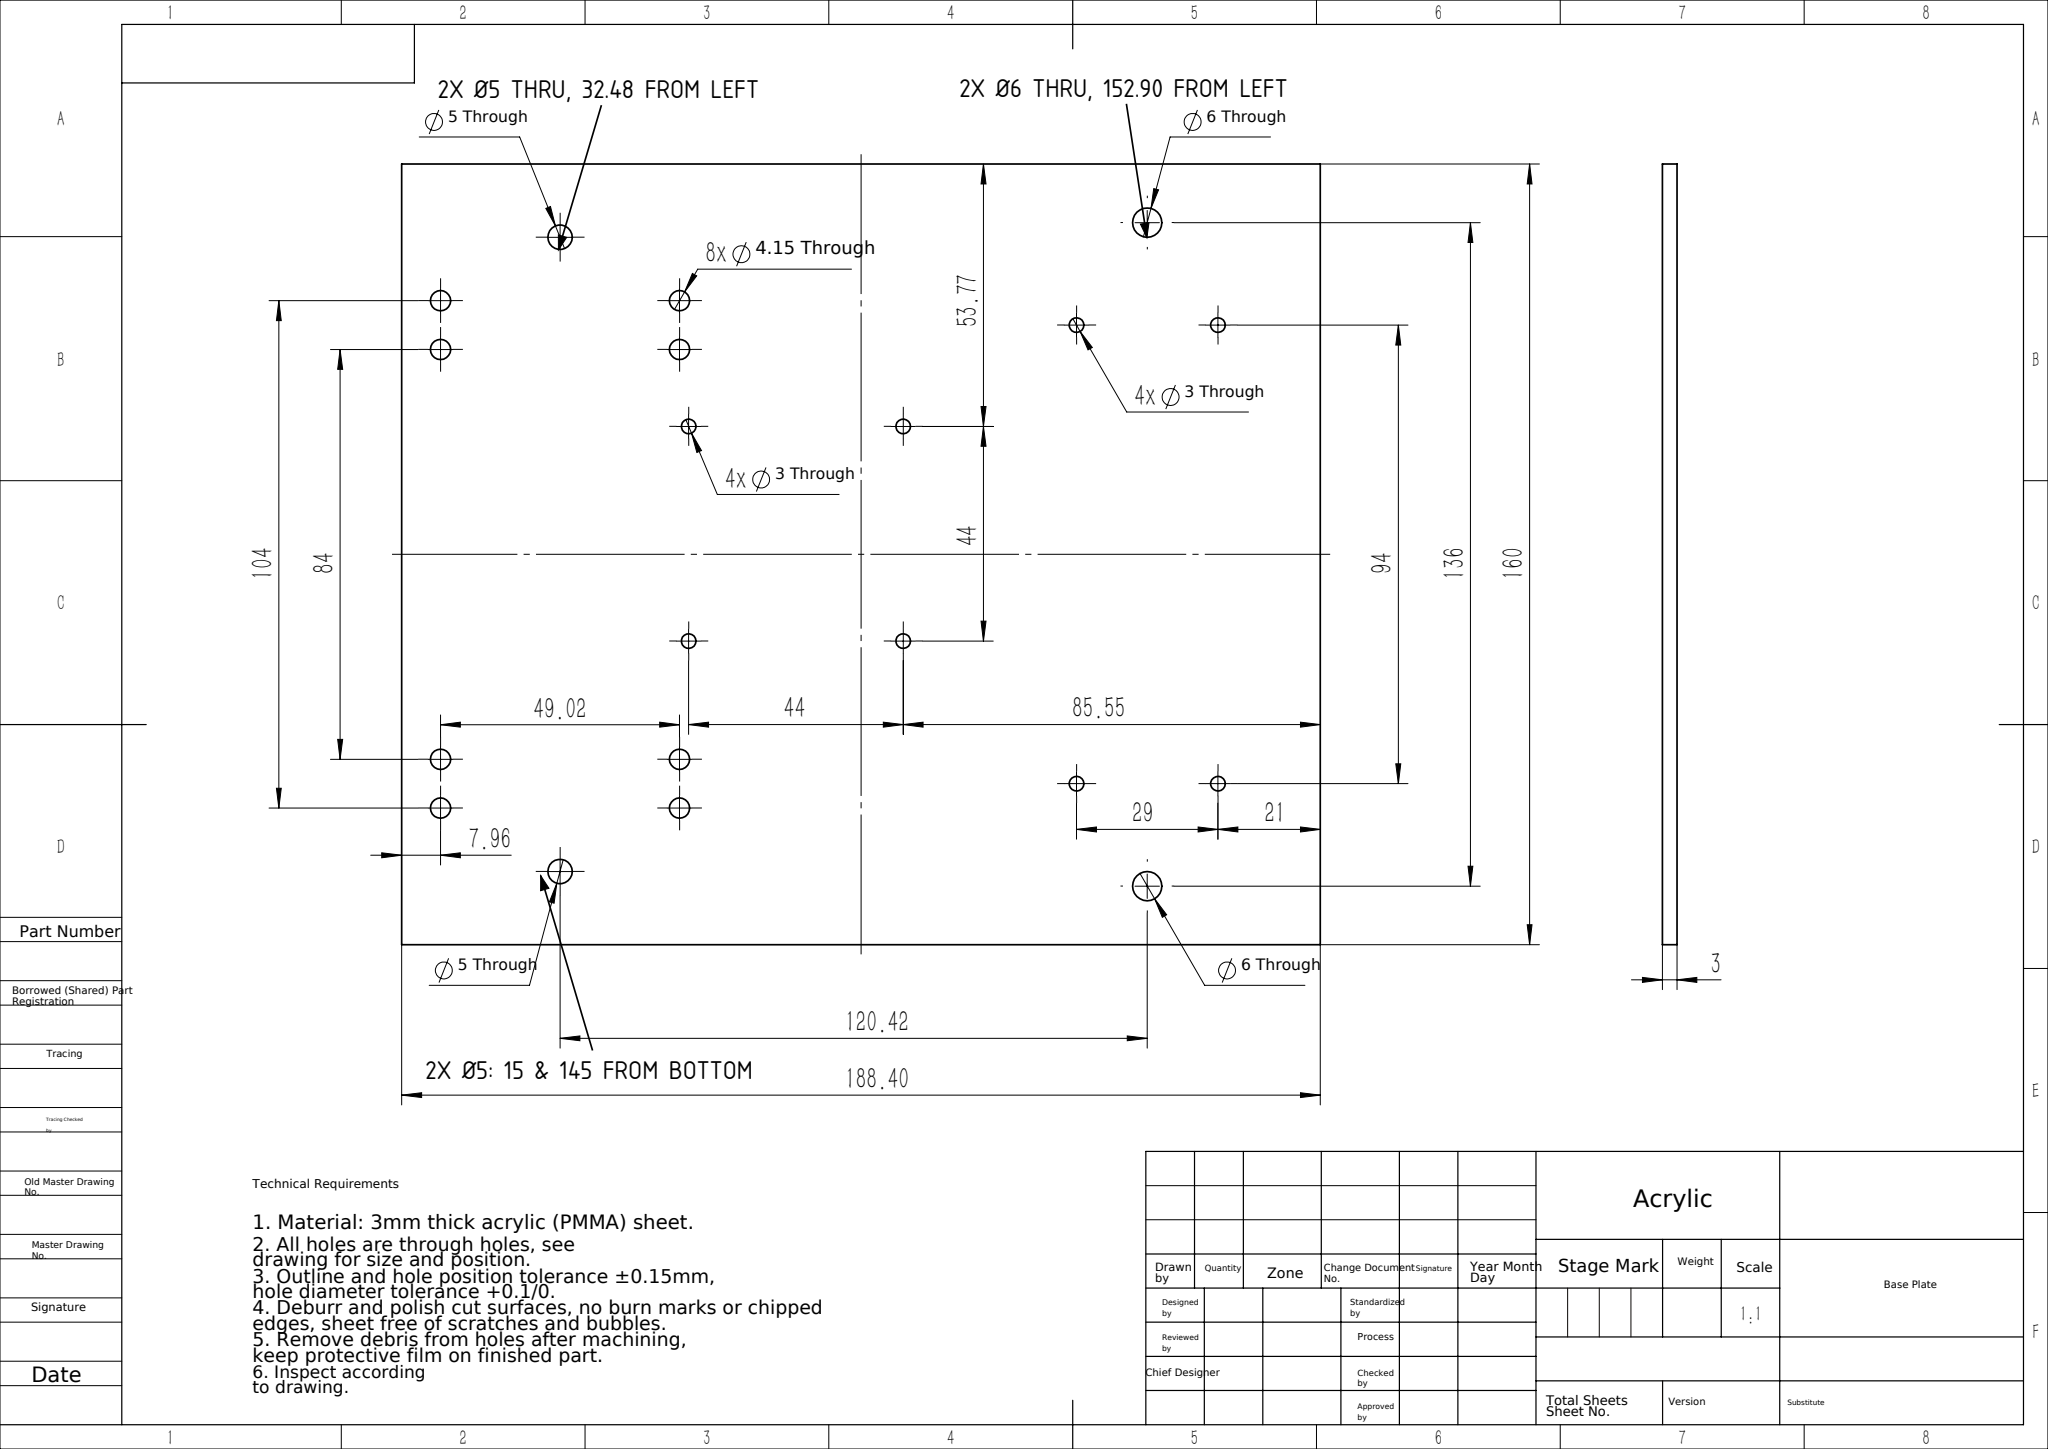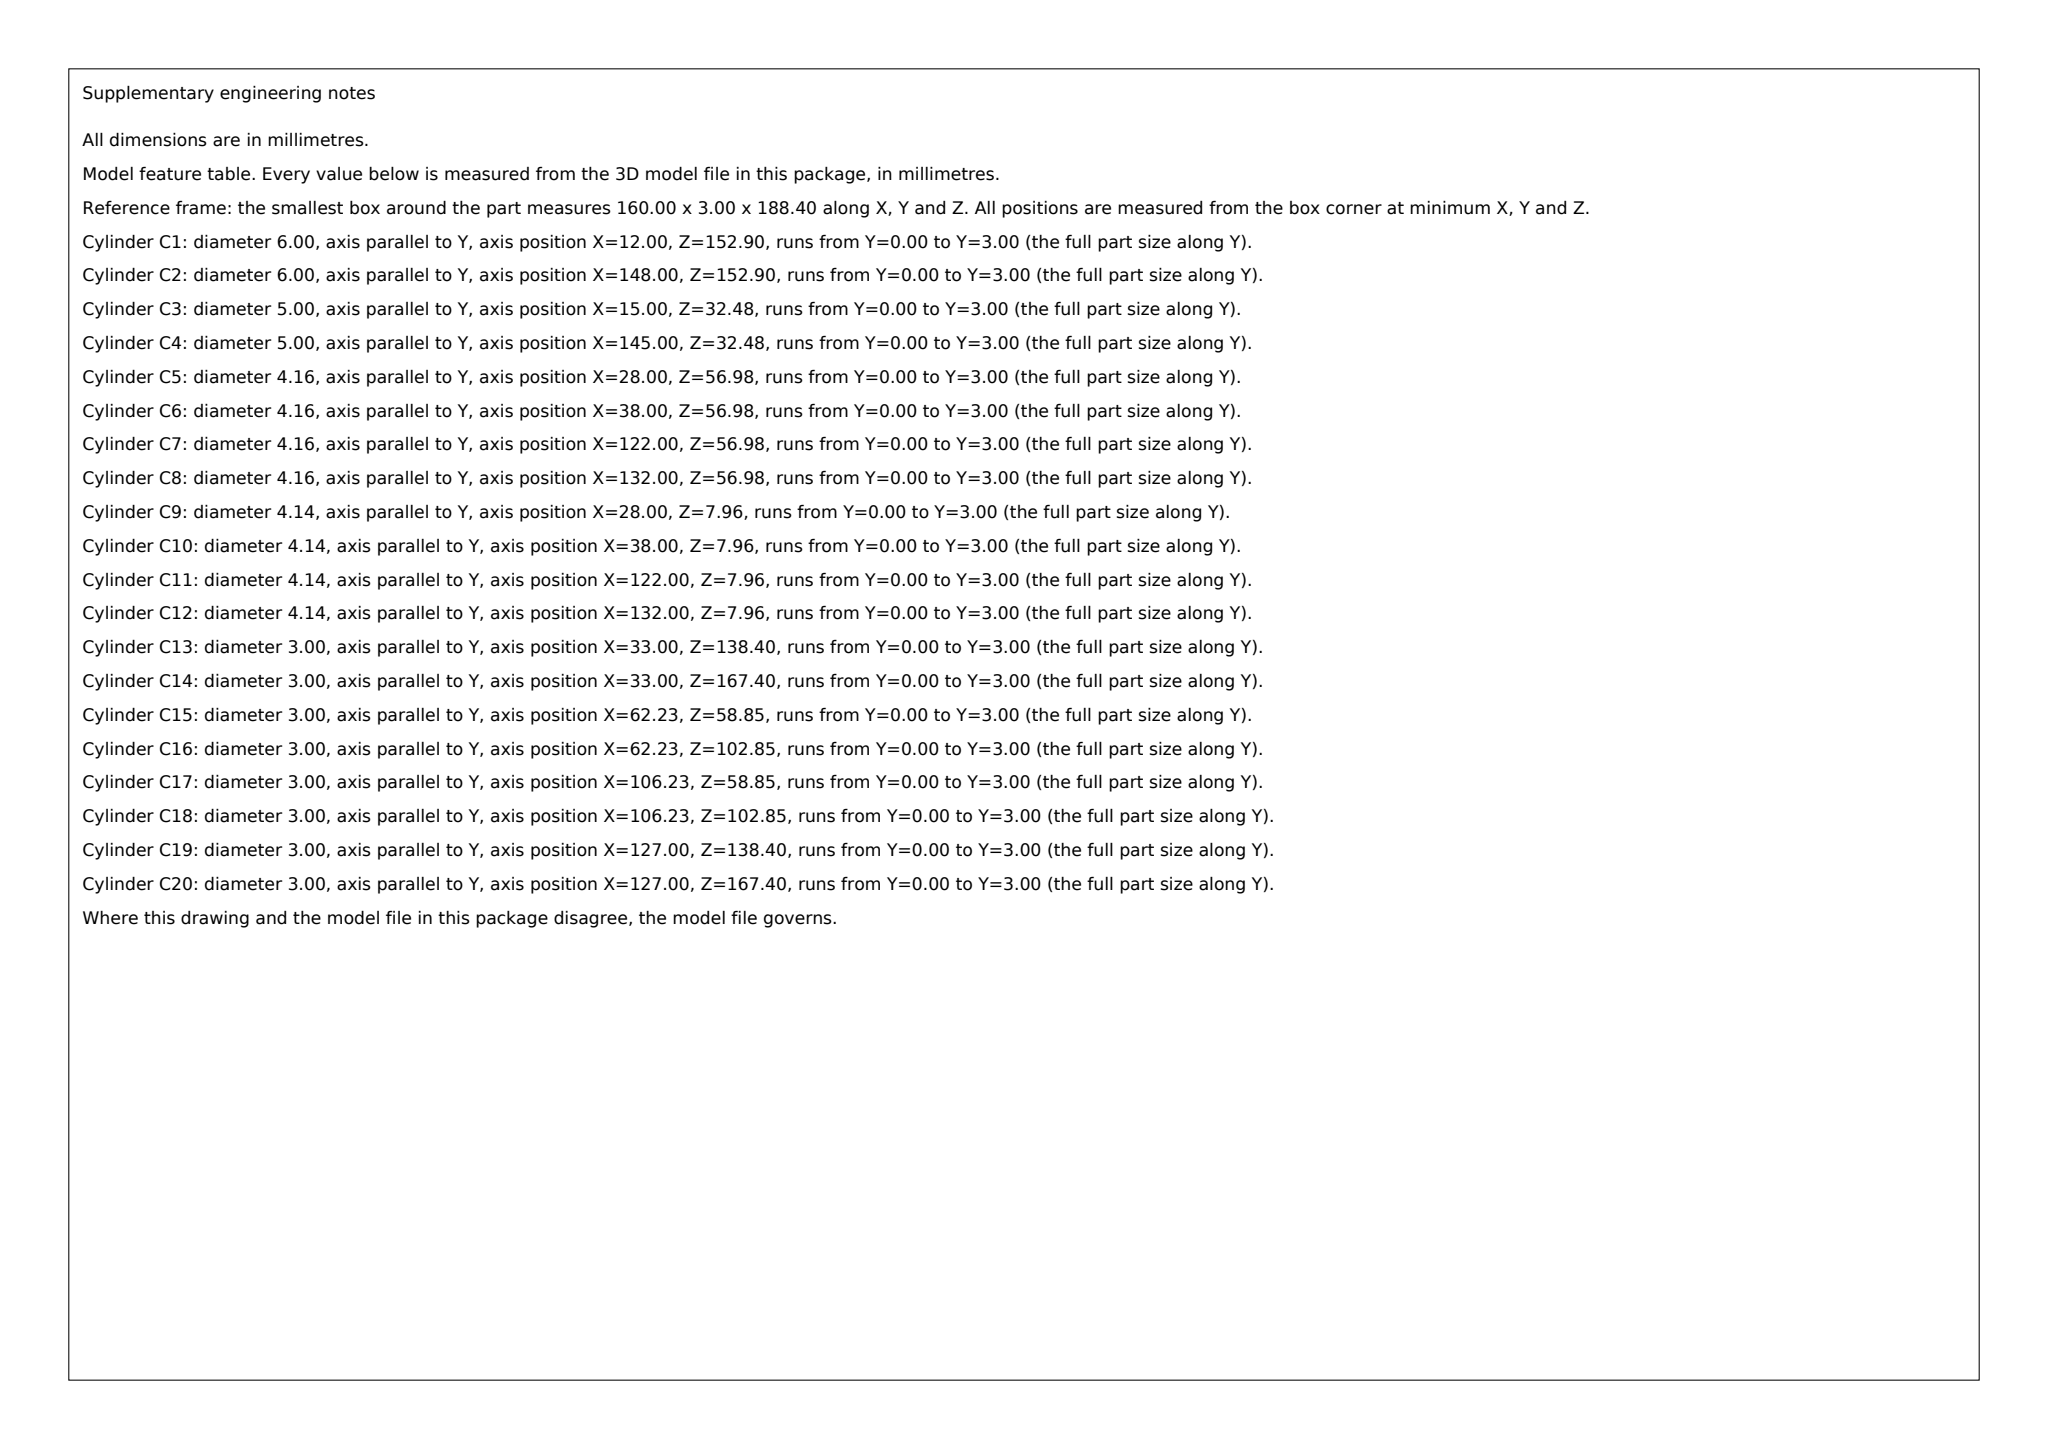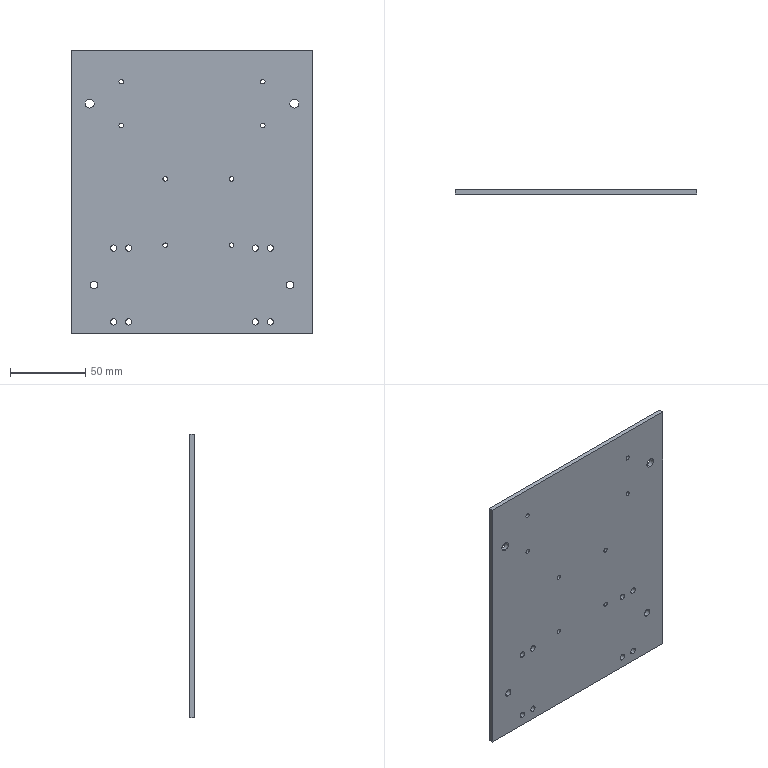Part | SolidWorks | mm | material PMMA | 1 solid | 46 faces | box 160 x 3 x 188.4 mm | volume 89648 mm3 | cylinder 40 | plane 6 | commonest cylinder face diameters 4.15 x16 3 x16 6 x4 5 x4
Drawing notes:
2X Ø5 THRU: hole centers located 32.48 mm from the left edge of the plate (188.40 side). | from the solid: cylinders dia 5.0, axis y, pos z = 32.48 (two holes), plate z-extent 0 to 188.4
2X Ø6 THRU: hole centers located 152.90 mm from the left edge of the plate (same datum as the 188.40 overall). | from the solid: cylinders dia 6.0, axis y, pos z = 152.9 (two holes), plate z-extent 0 to 188.4
2X Ø5 THRU: hole centers 15 mm and 145 mm from the bottom edge (160 side), i.e. 130 mm apart, symmetric about the horizontal centerline (±65). | from the solid: cylinders dia 5.0, axis y, pos x = 15.0 and 145.0, plate x-extent 0 to 160.0